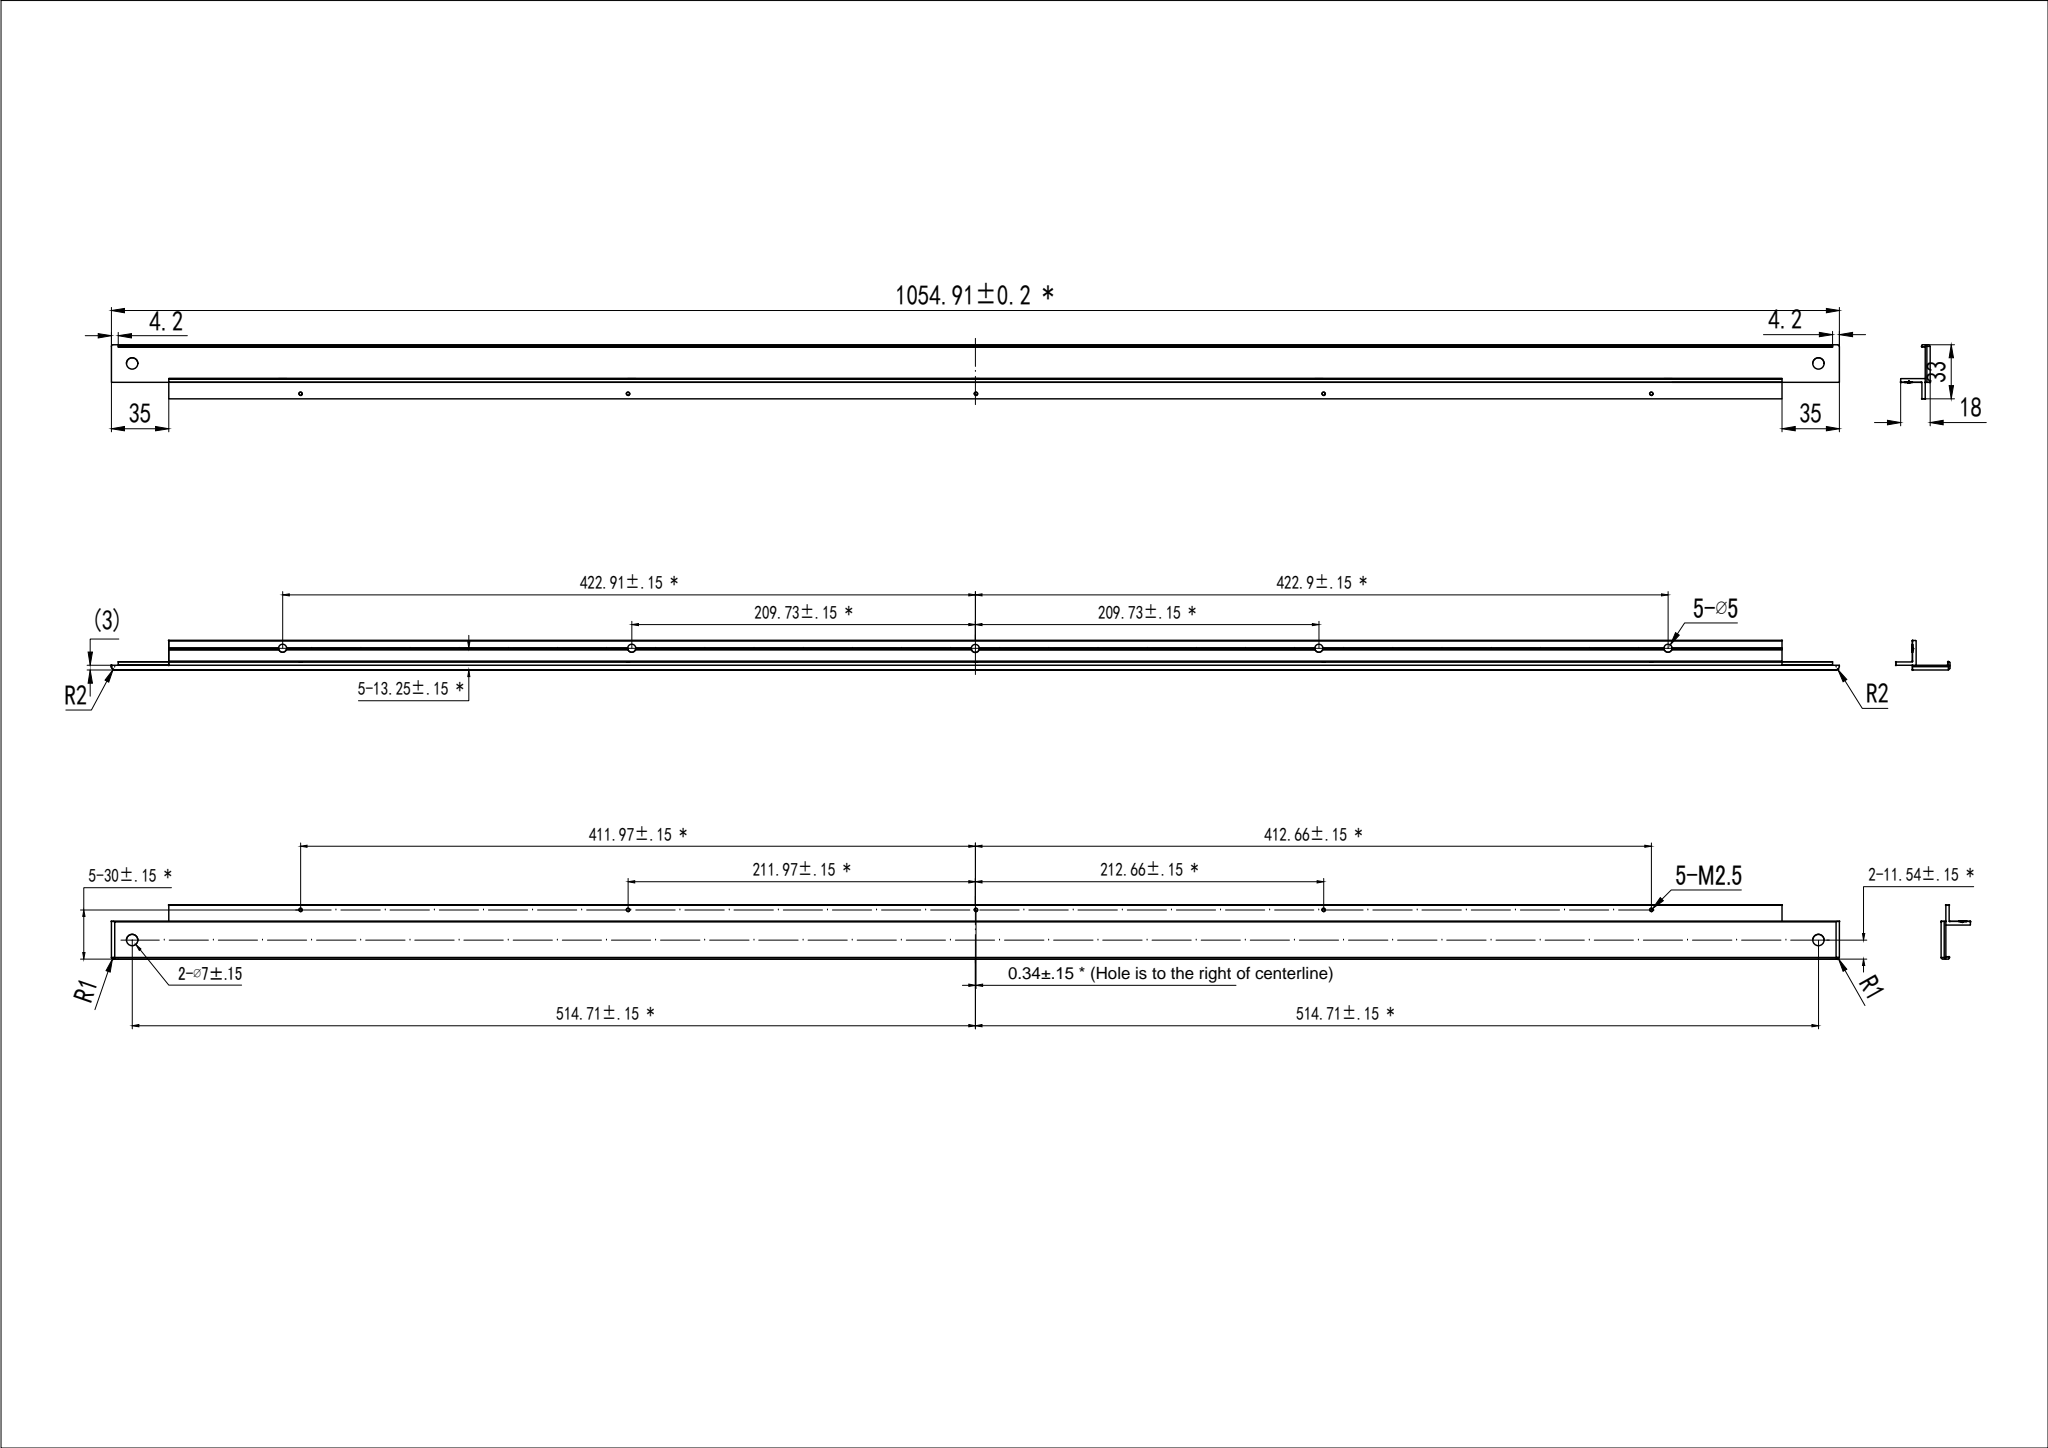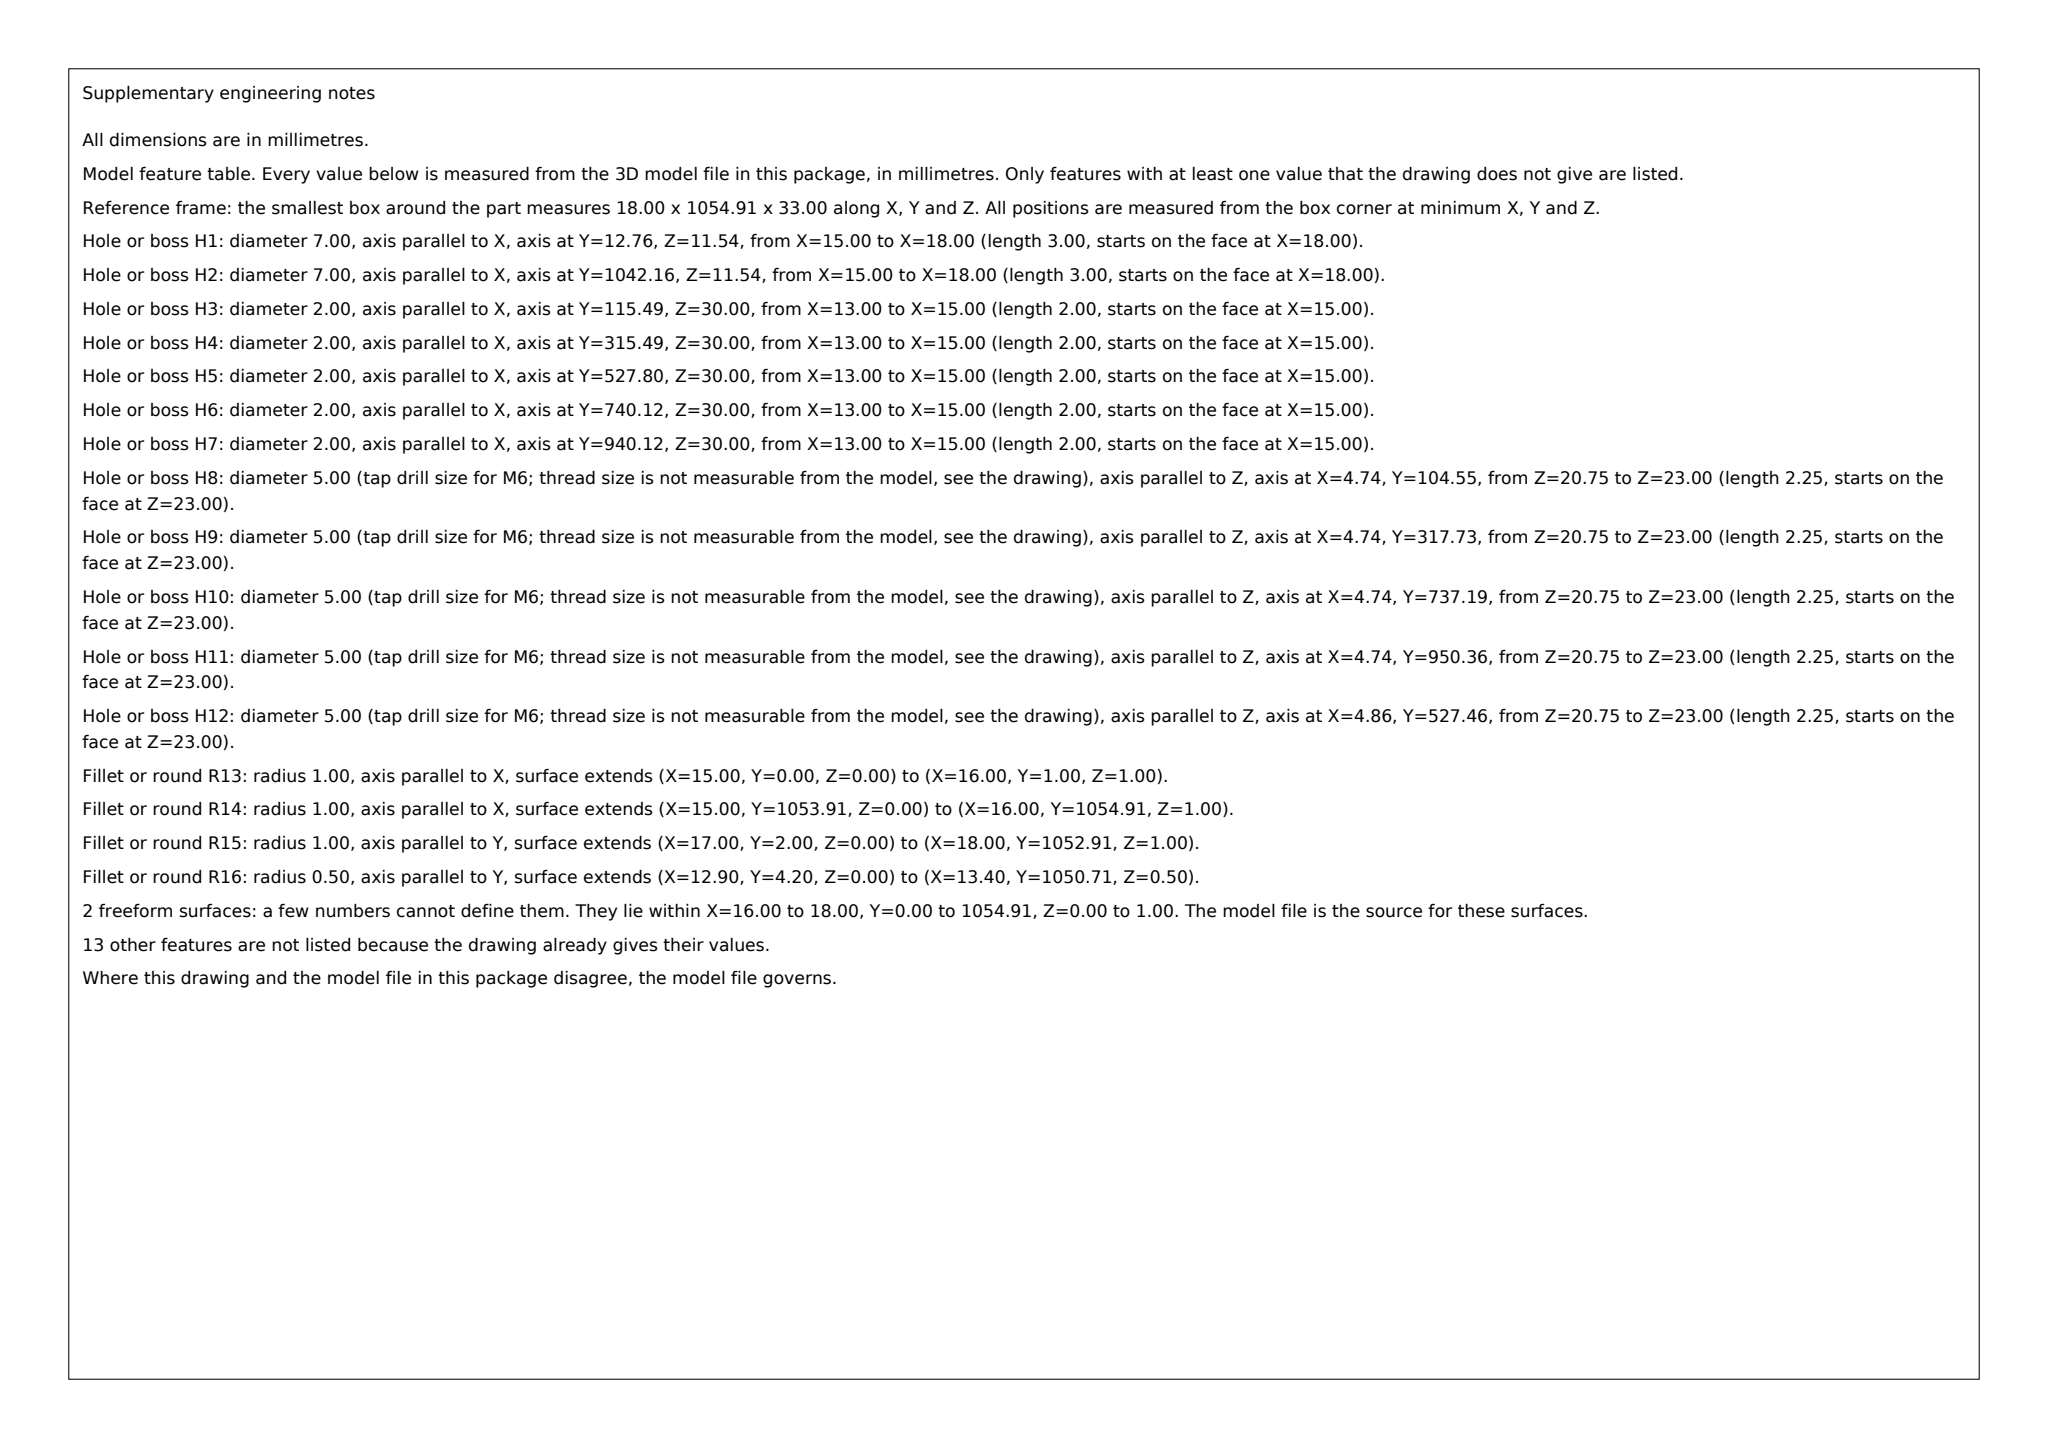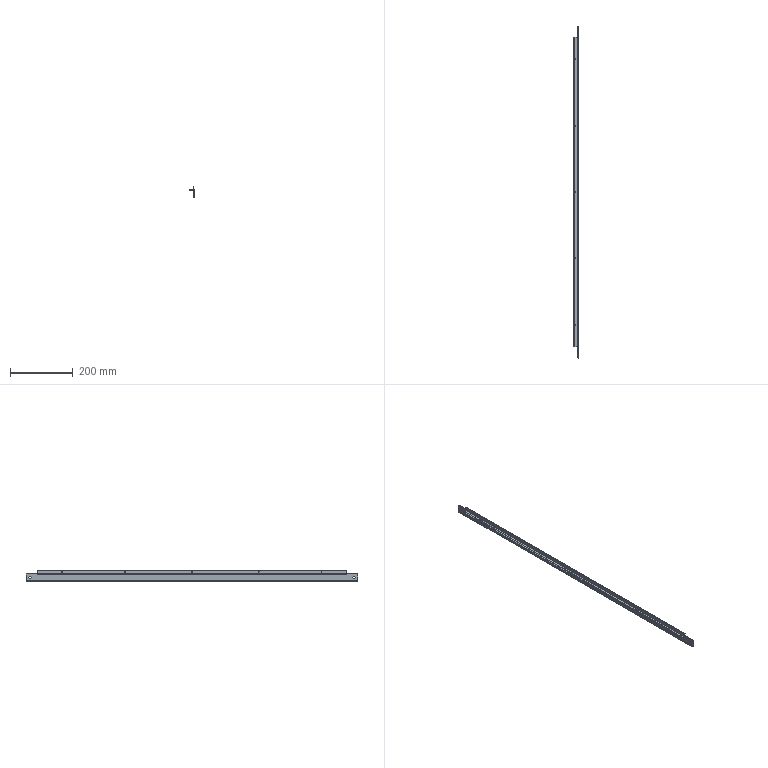Part | SolidWorks | mm | 1 solid | 88 faces | box 18 x 1054.91 x 33 mm | volume 127527 mm3 | cylinder 54 | plane 32 | spline 2 | commonest cylinder face diameters 0.4 x24 2 x13 5 x10 7 x4 4 x2 1 x1